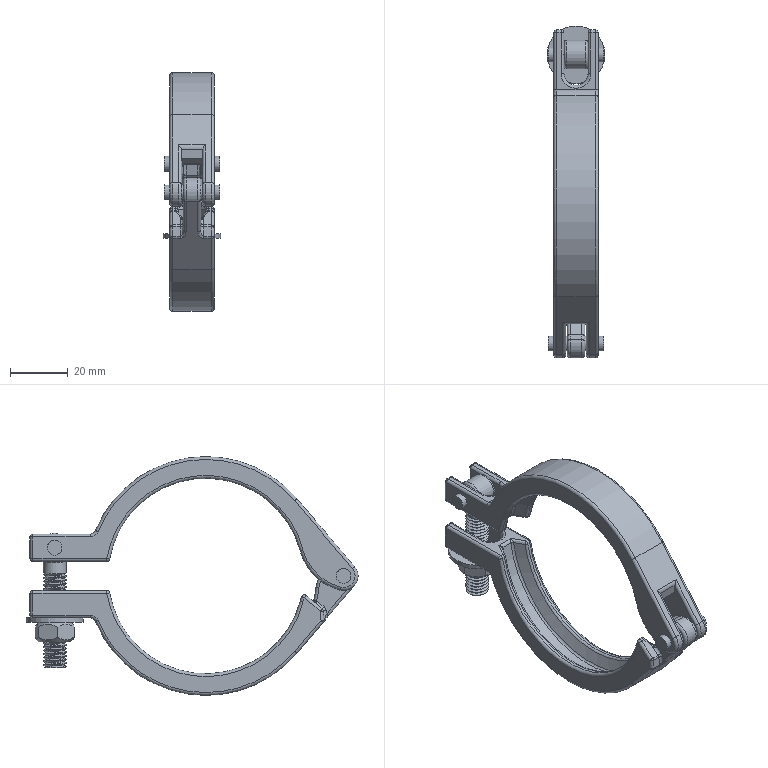Assembly | NX | mm | 7 component files | 7 solids | 311 faces | box 20 x 114.75 x 82.5 mm | volume 26316 mm3 | cylinder 124 | spline 51 | torus 48 | plane 46 | sphere 34 | cone 8 | commonest cylinder face diameters 2 x61 7.94 x27 5.1 x7 38.209 x5 10 x4 67.5 x4 4 x3 20 x2
Bill of materials:
unnamed part 1 | 1 |  | Hexagonal nut: a six-sided prism with chamfered corners at both ends and a central threaded through-bore.
unnamed part 2 | 1 |  | Eye bolt / eye screw: a cylindrical ring eye with a through-hole on top of a short plain neck and a long externally threaded shank.
unnamed part 3 | 2 |  | Plain solid cylinder (round rod or pin) with flat ends and no visible features.
unnamed part 4 | 1 |  | Flat washer: a thin annular disc with a concentric central through-hole.
unnamed part 5 | 1 |  | Curved arm or half-clamp segment. A roughly semicircular arc band has a recessed channel on its concave inner face. One end is a straight forked tab with a U-shaped notch between two prongs. The other end is a narrower angled lug with a single round hole, separated from the arc by a small stepped notch.
unnamed part 6 | 1 |  | Arched arm with clevis-style forked ends. A curved arch band has two-prong forks at both ends, each prong with a cross hole. One end is a straight offset tab and the other an angled tail. A small rectangular pocket or step is under the arch near the straight end.
Mates:
1. fix | top_buckle 1 component
2. align lock | pin 2 face | top_buckle 1 face
3. distance | pin 2 face | top_buckle 1 face
4. align lock | bolt 1 face | pin 2 face
5. touch align | bolt 1 face | top_buckle 1 face
6. align lock | bottom_buckle 1 face | top_buckle 1 face
7. touch align | bottom_buckle 1 face | top_buckle 1 face
8. align lock | washer 1 face | bolt 1 face
9. touch align | nut 1 face | washer 1 face
10. touch align | washer 1 face | bottom_buckle 1 face
11. align lock | pin 1 face | top_buckle 1 face
12. distance | pin 1 face | top_buckle 1 face